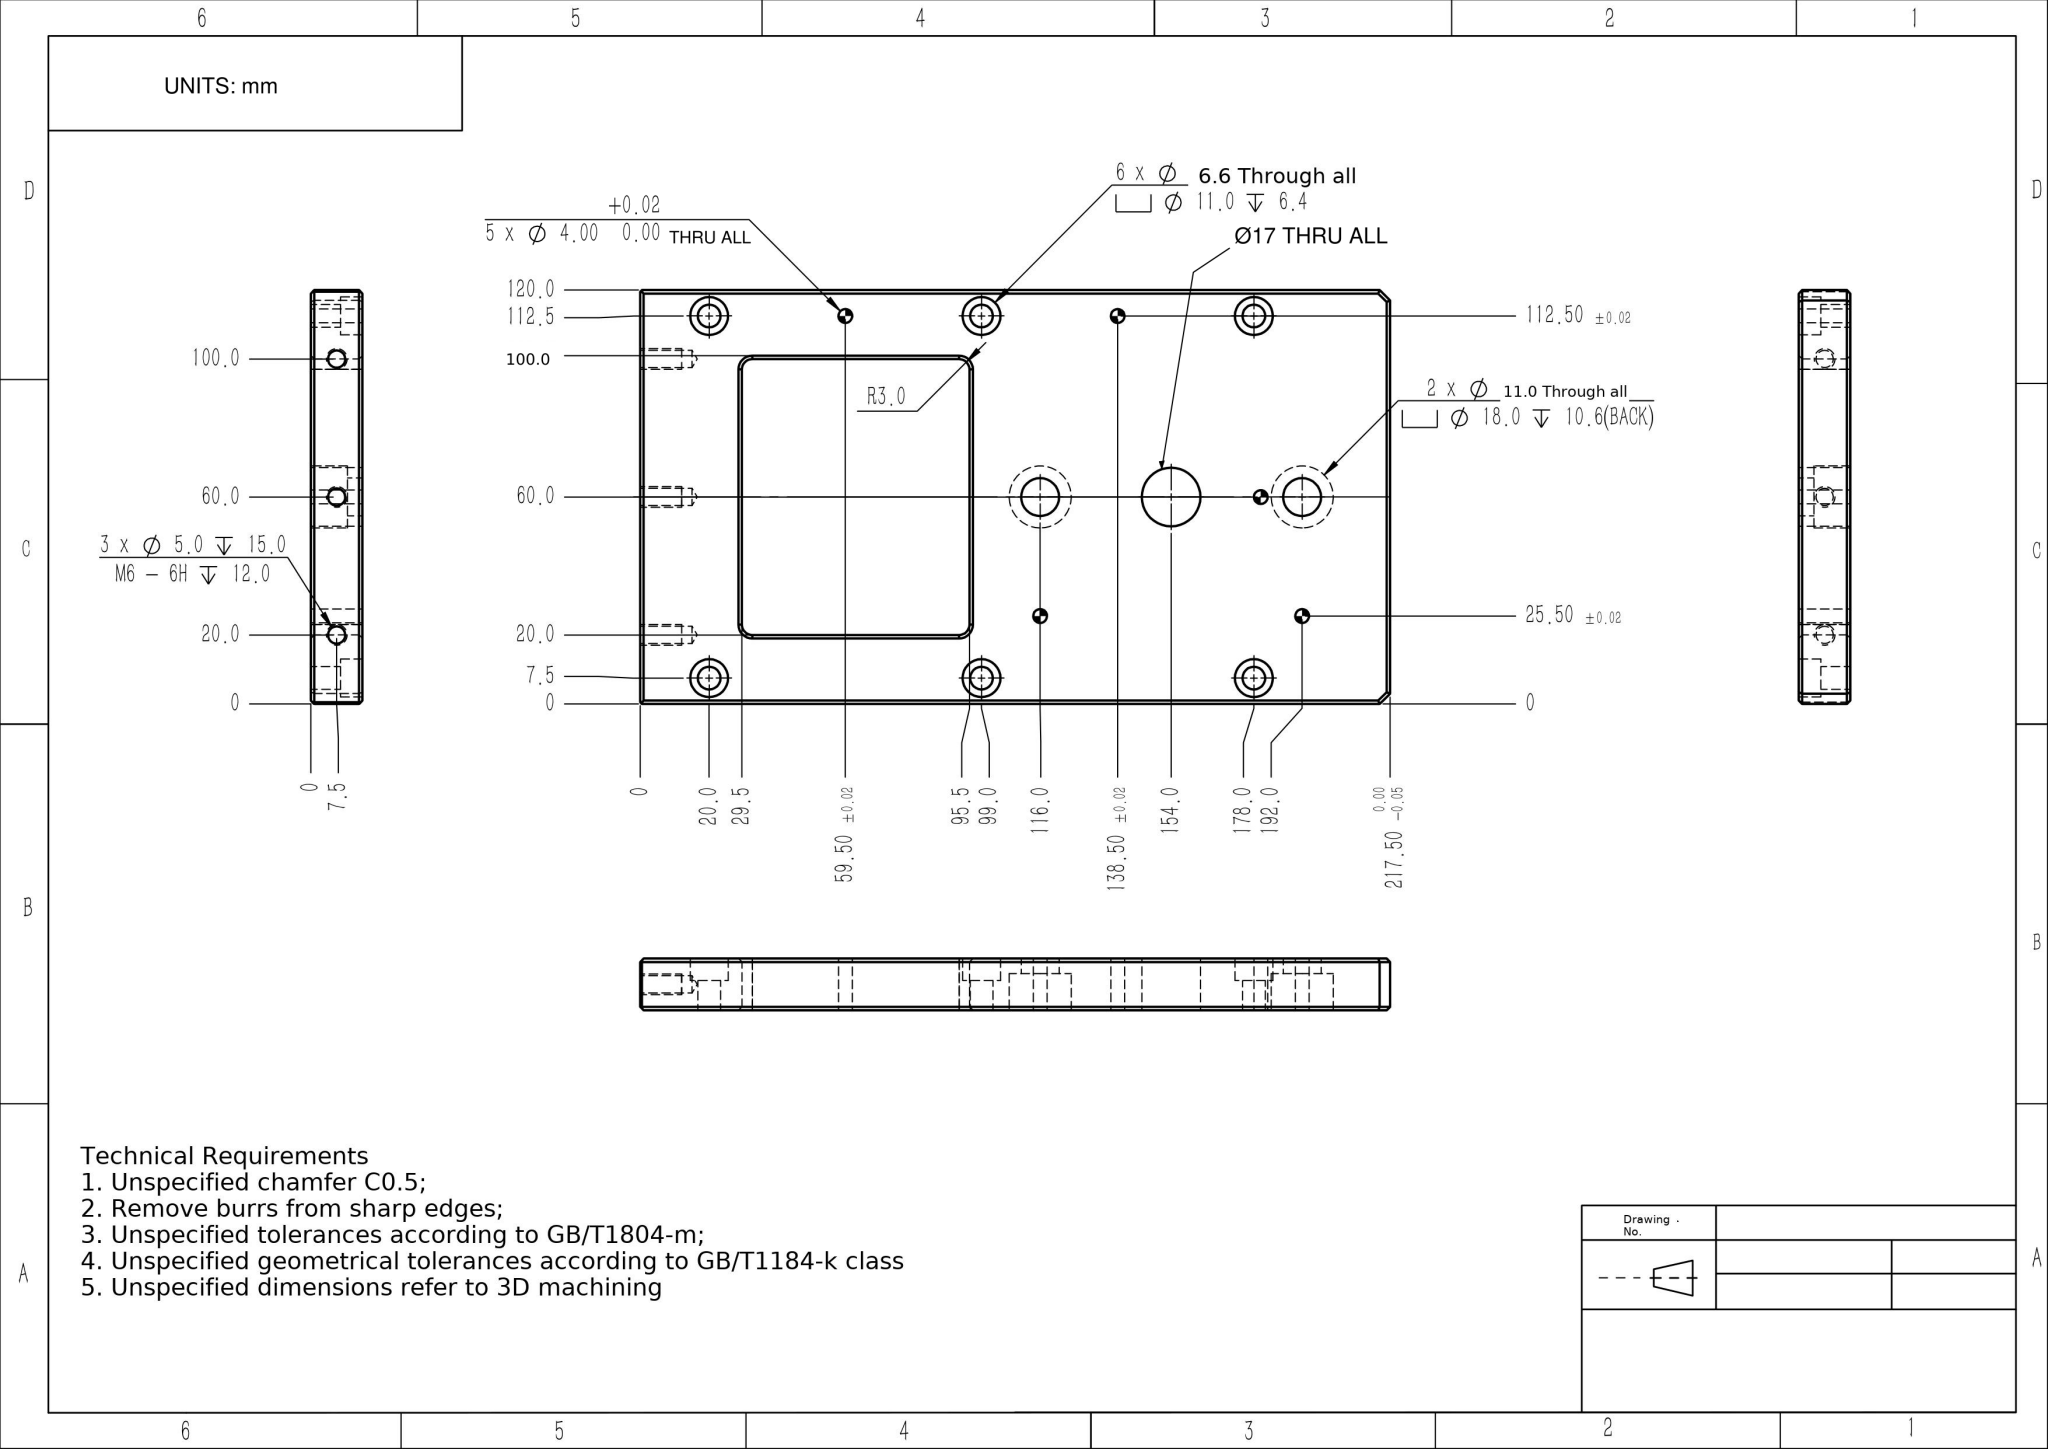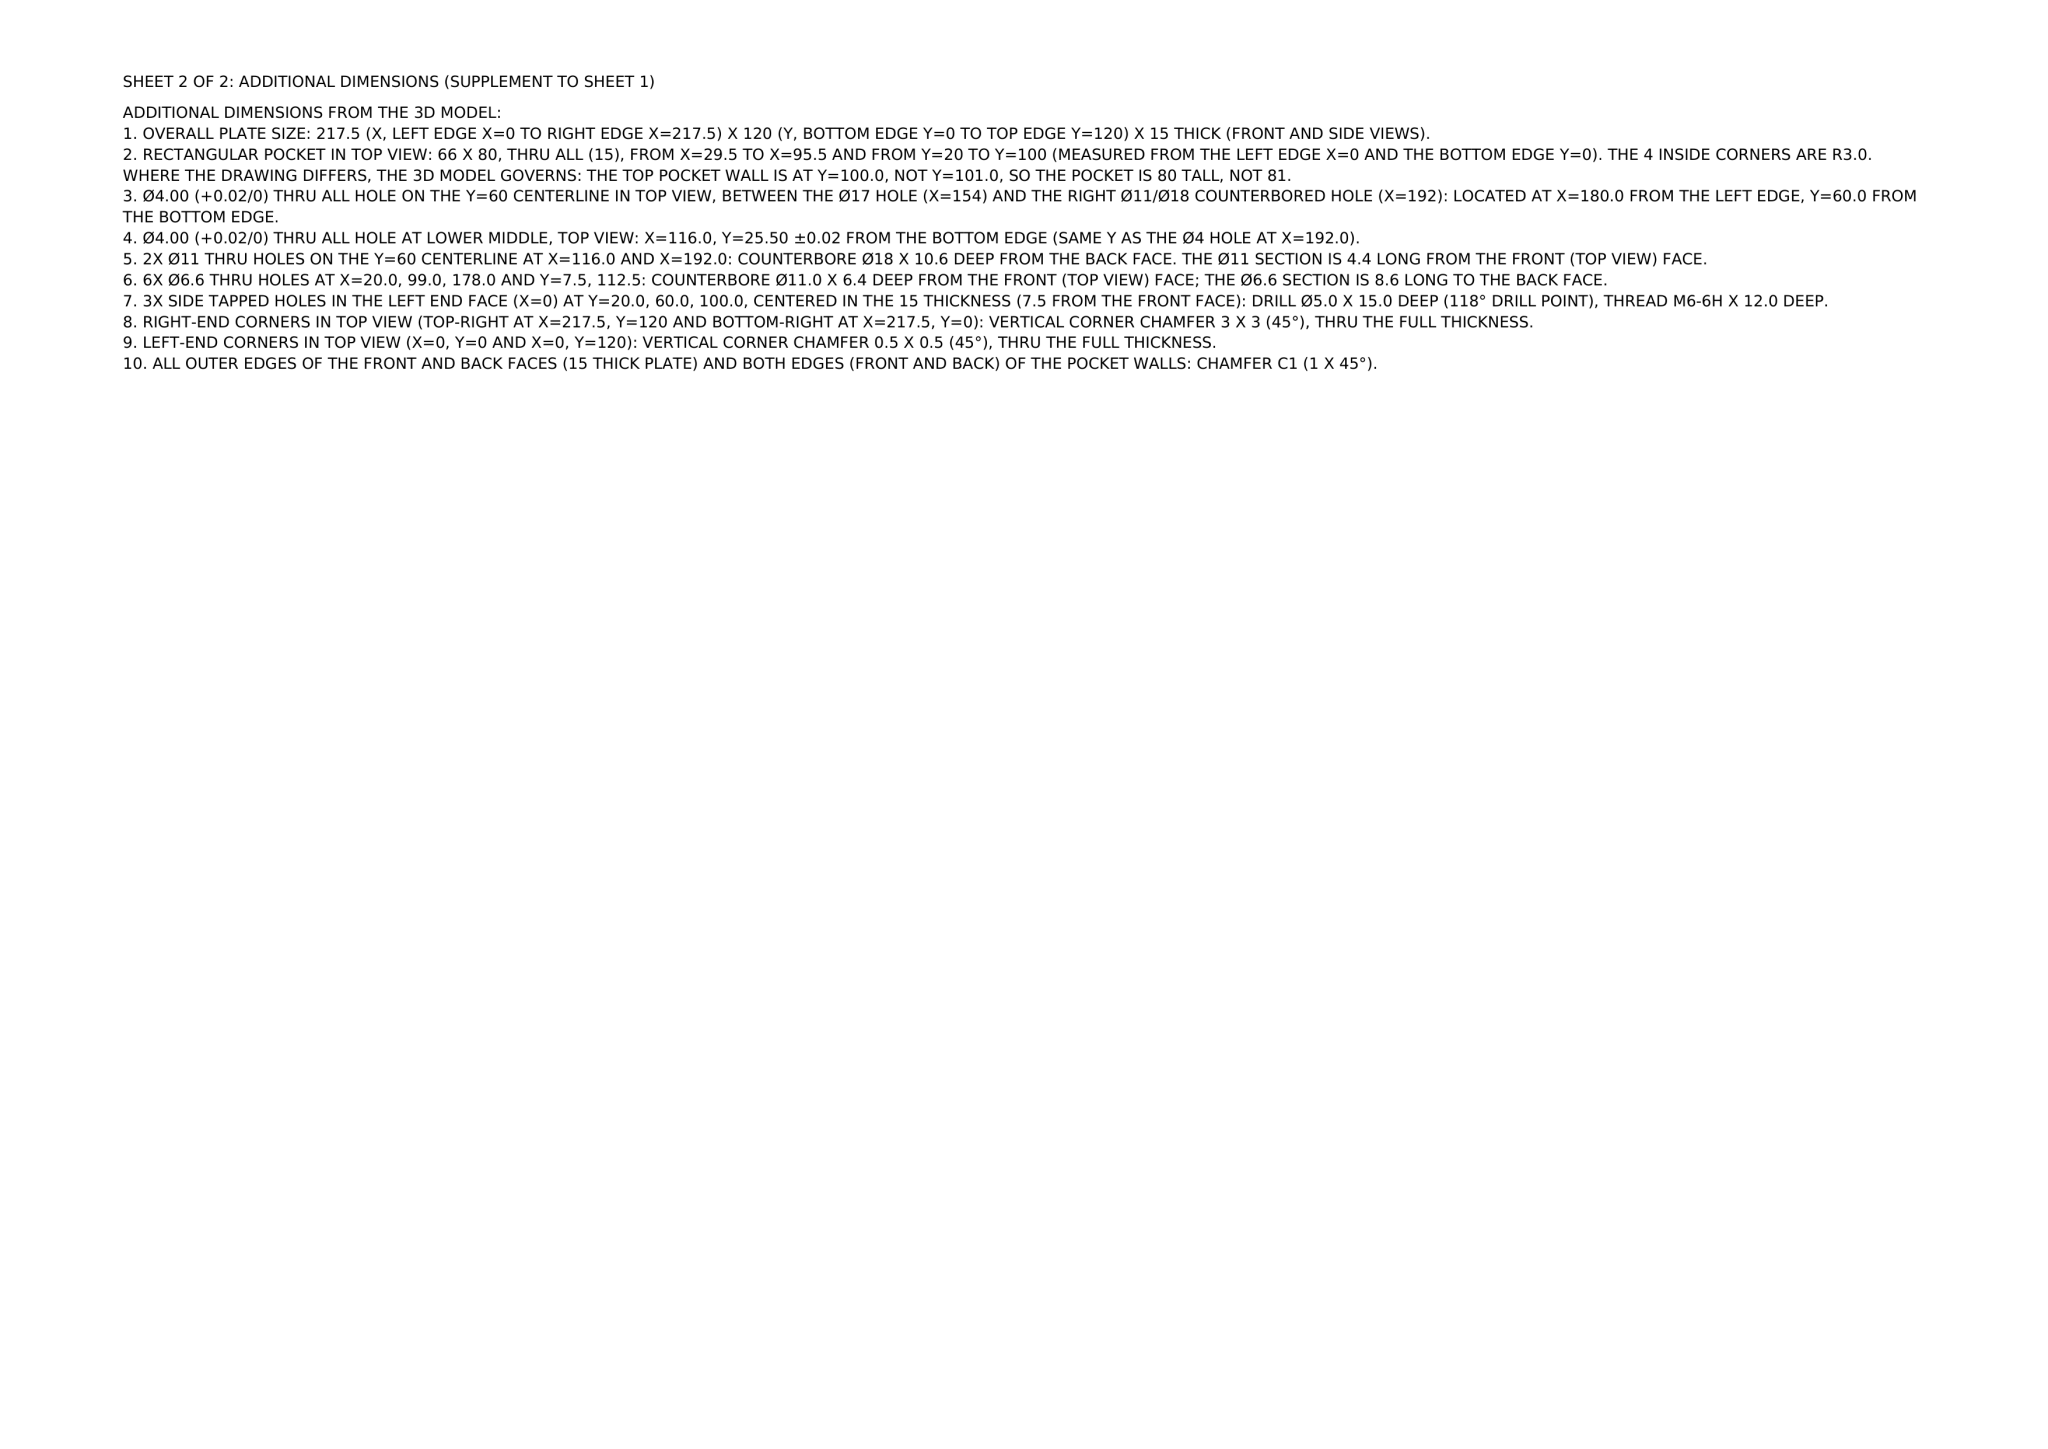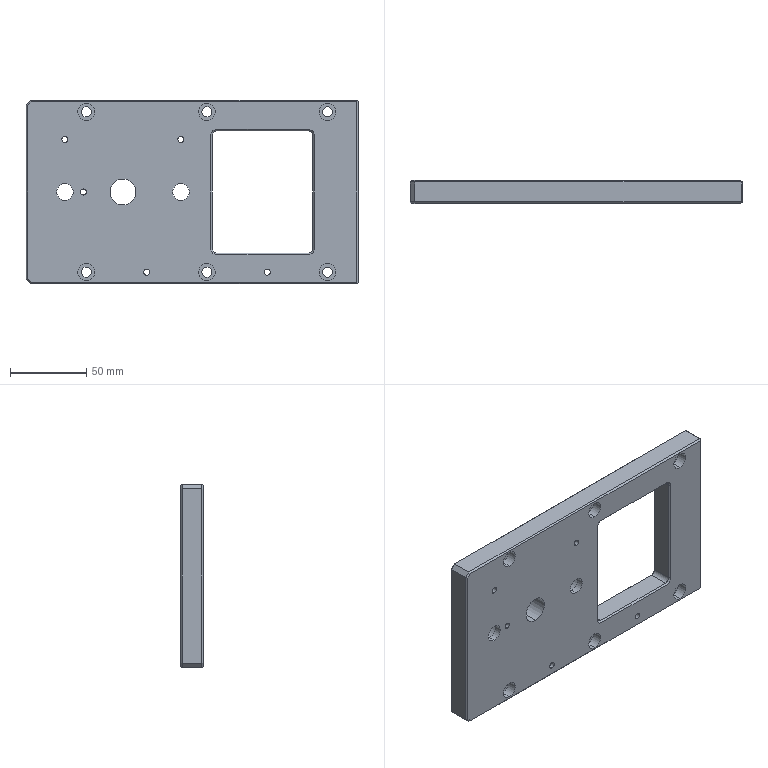Part | NX | mm | 1 solid | 110 faces | box 217.5 x 15 x 120 mm | volume 294414 mm3 | cylinder 54 | plane 42 | cone 14 | commonest cylinder face diameters 11 x16 6.6 x12 4 x10 5 x6 18 x4 6 x4 17 x2